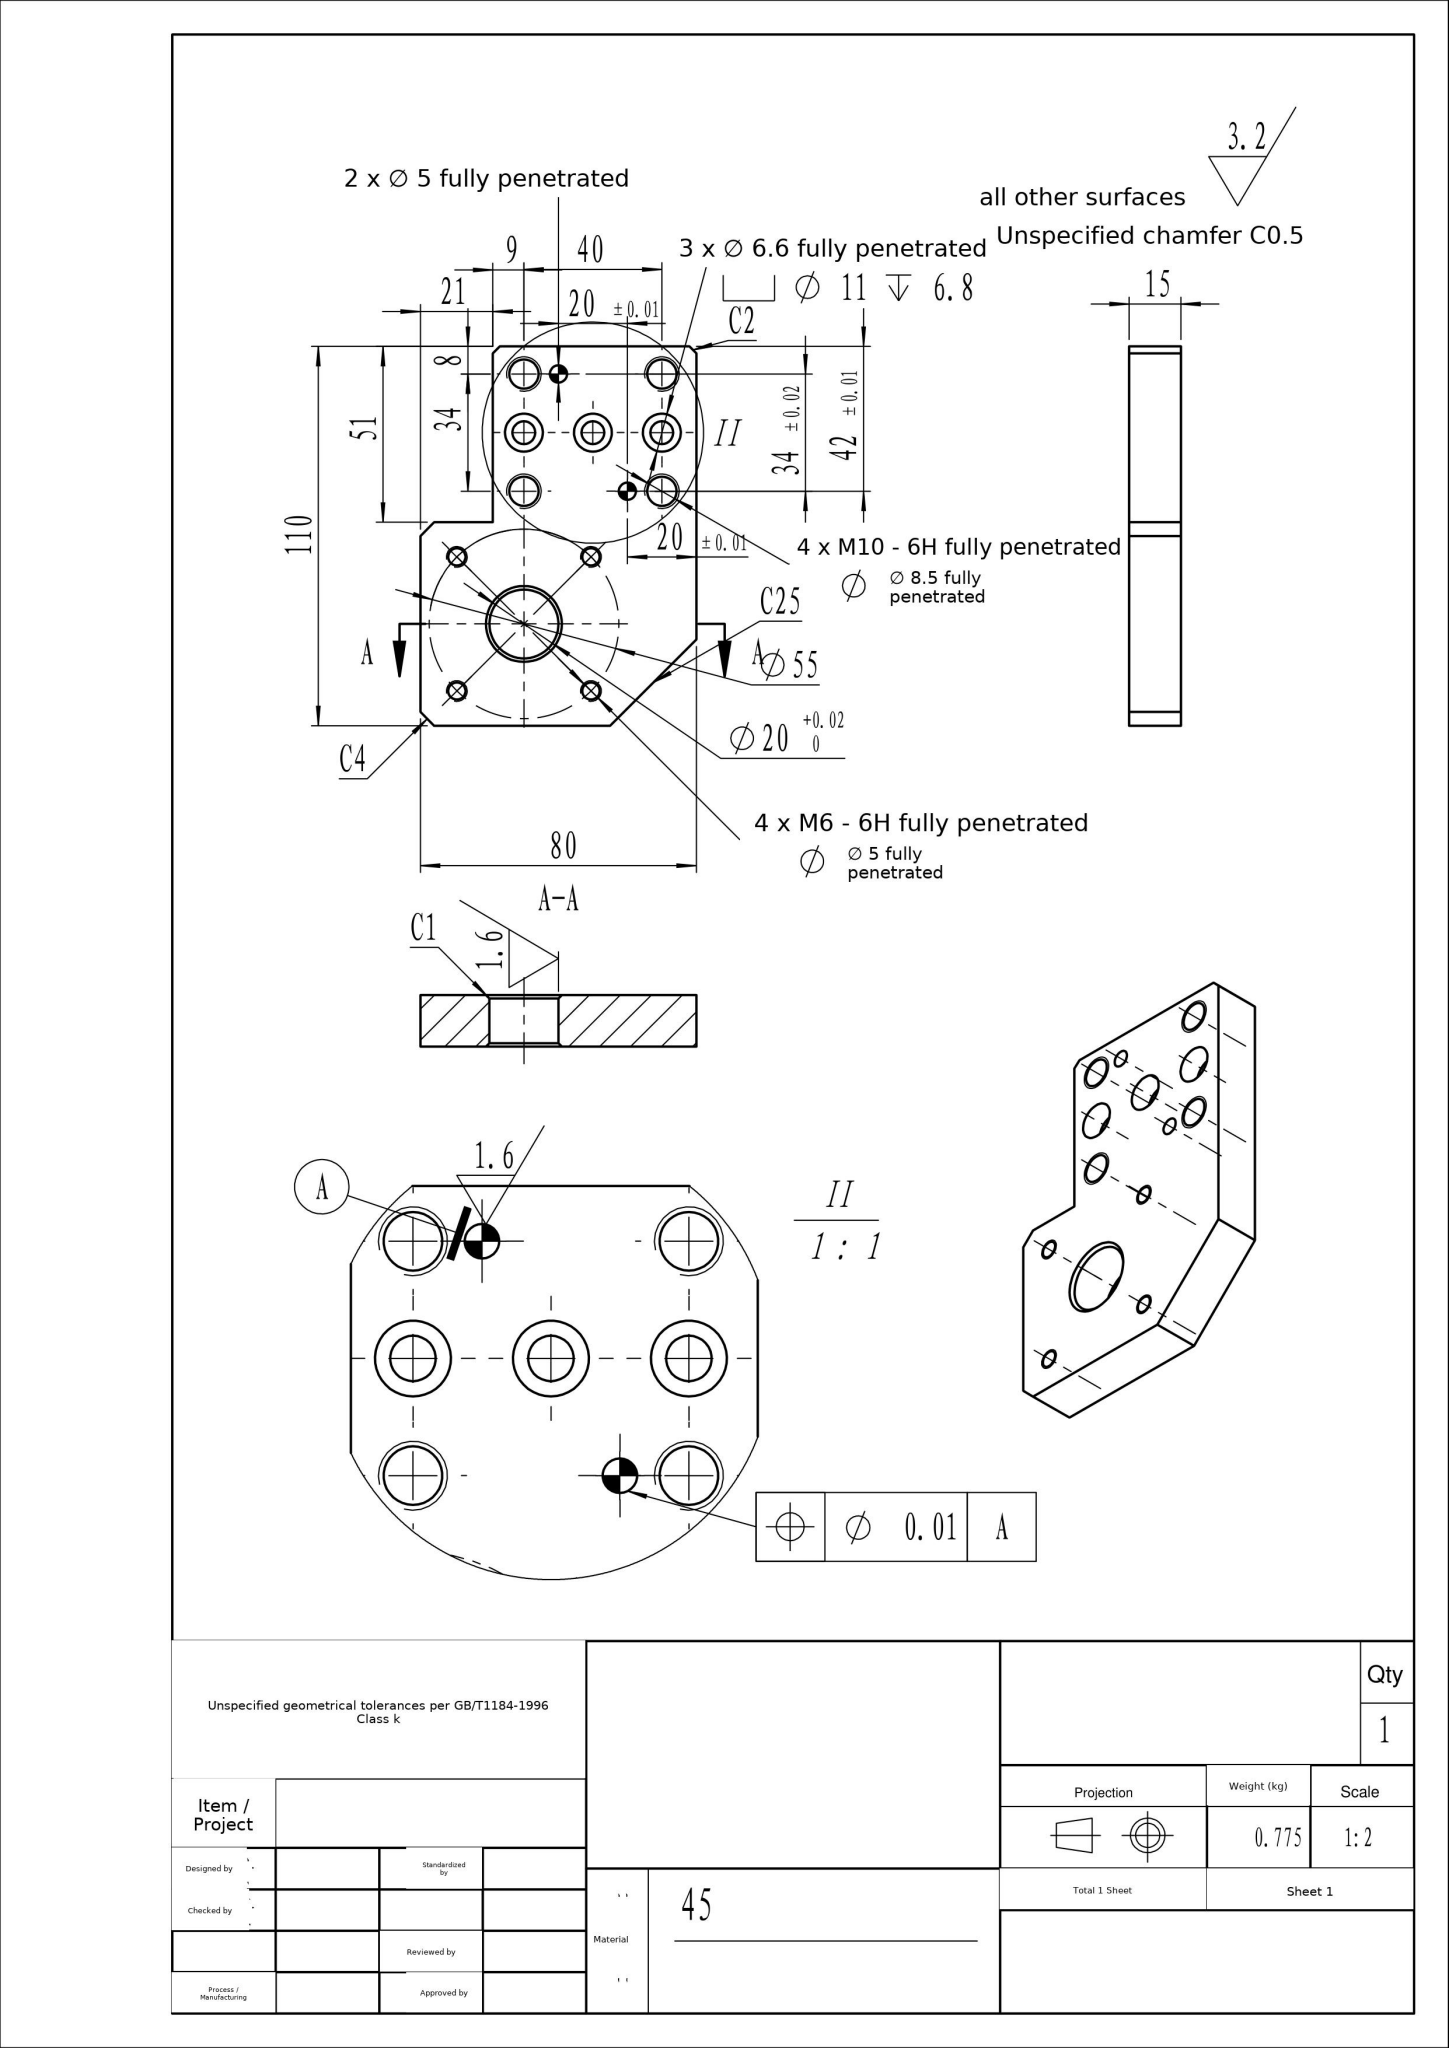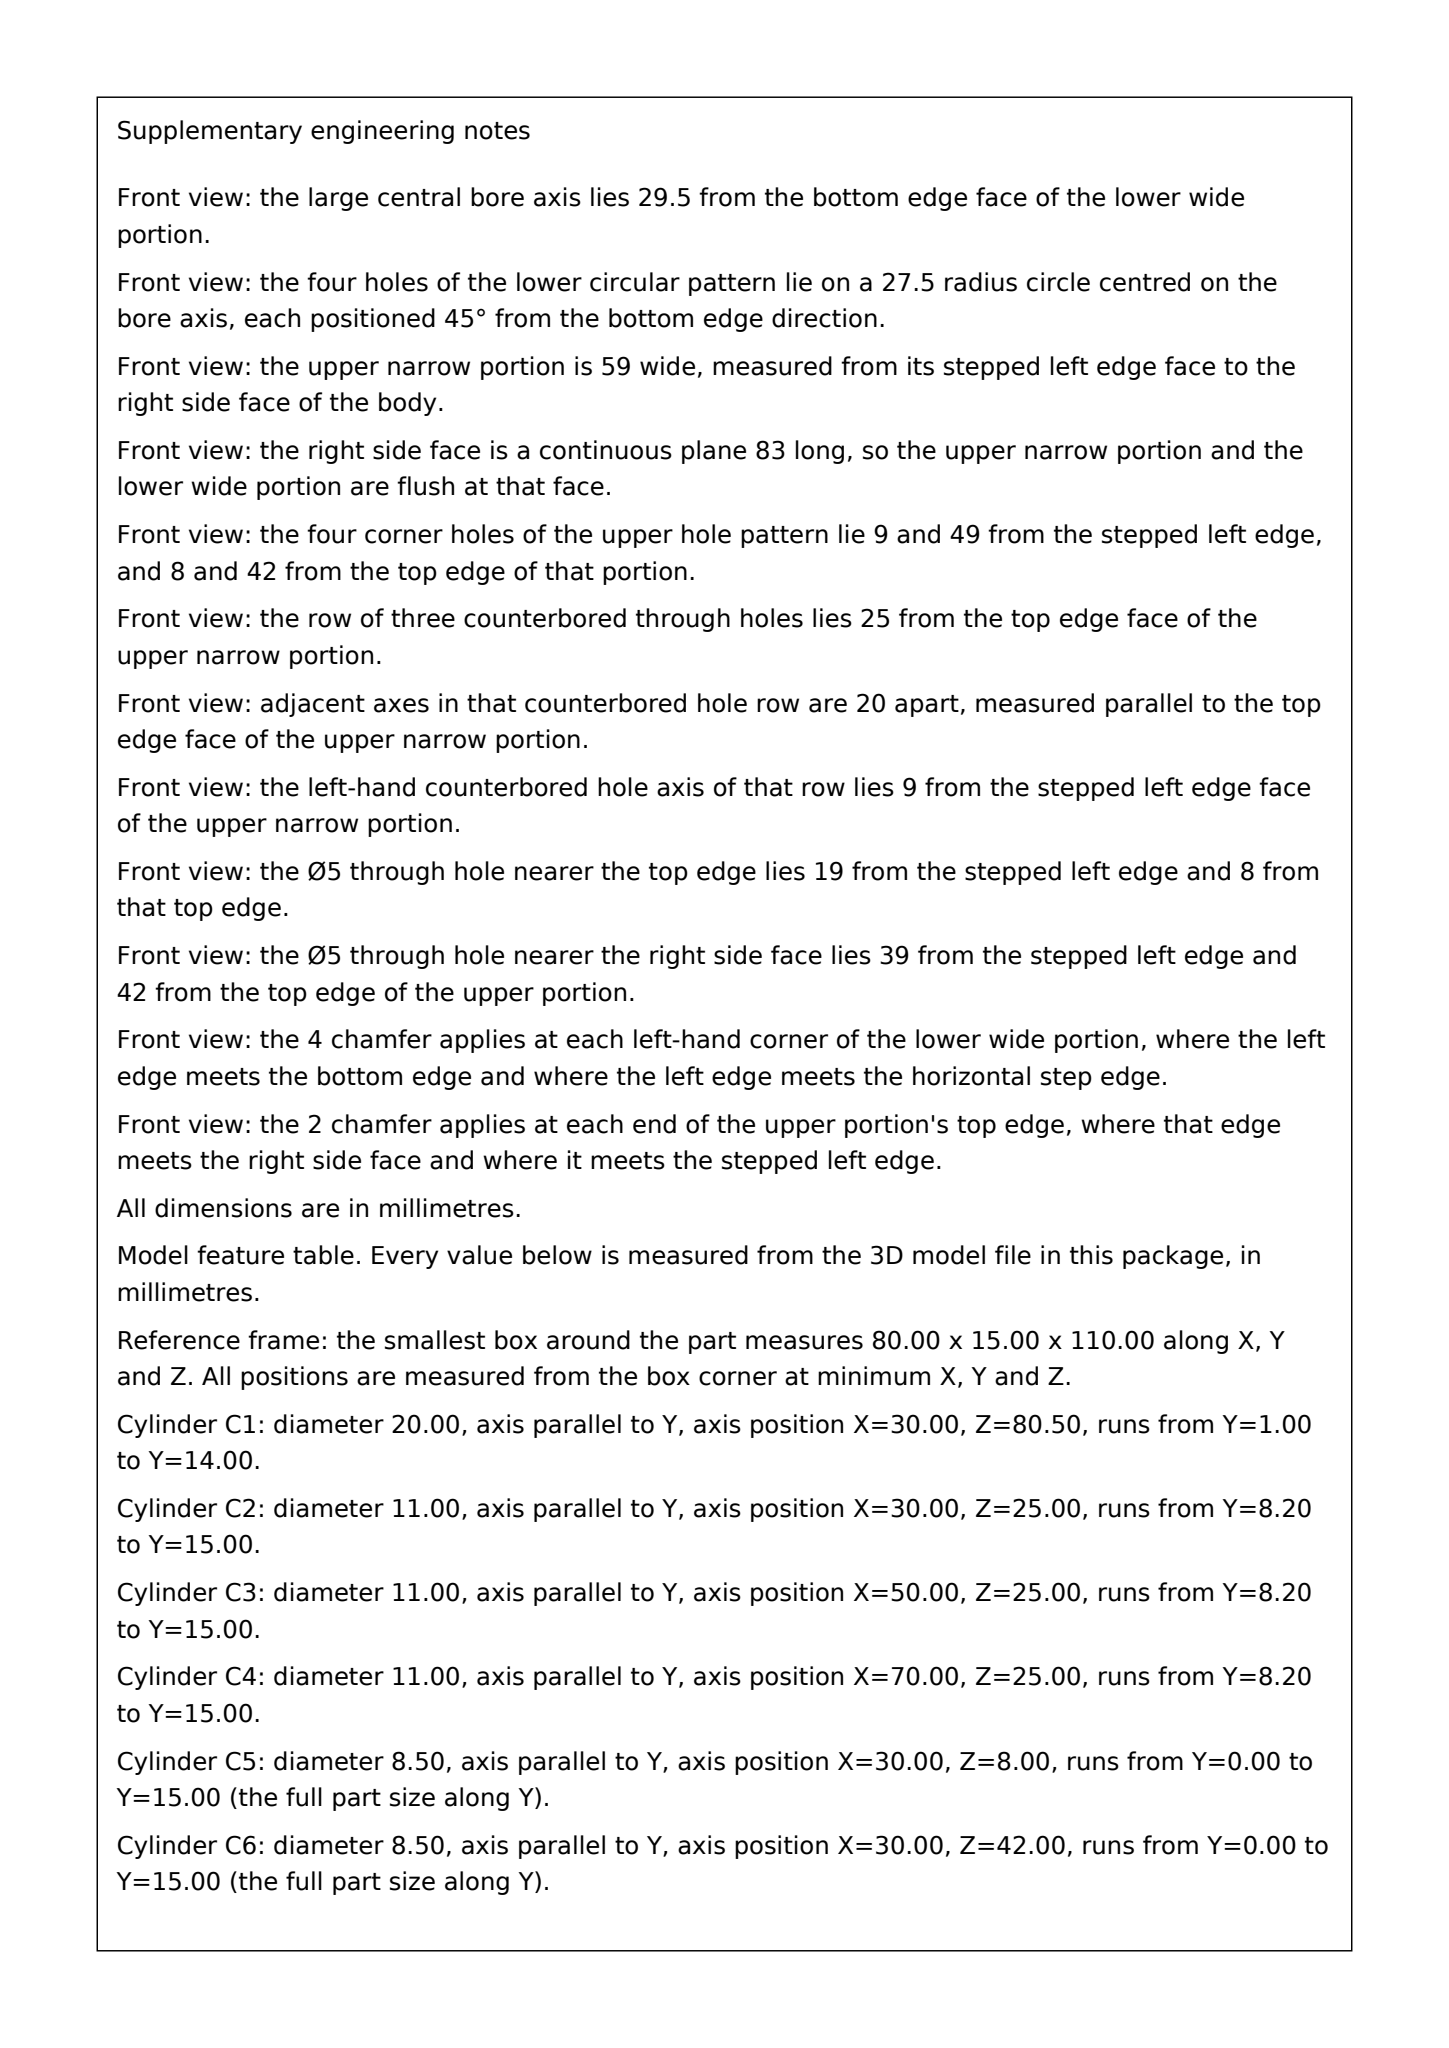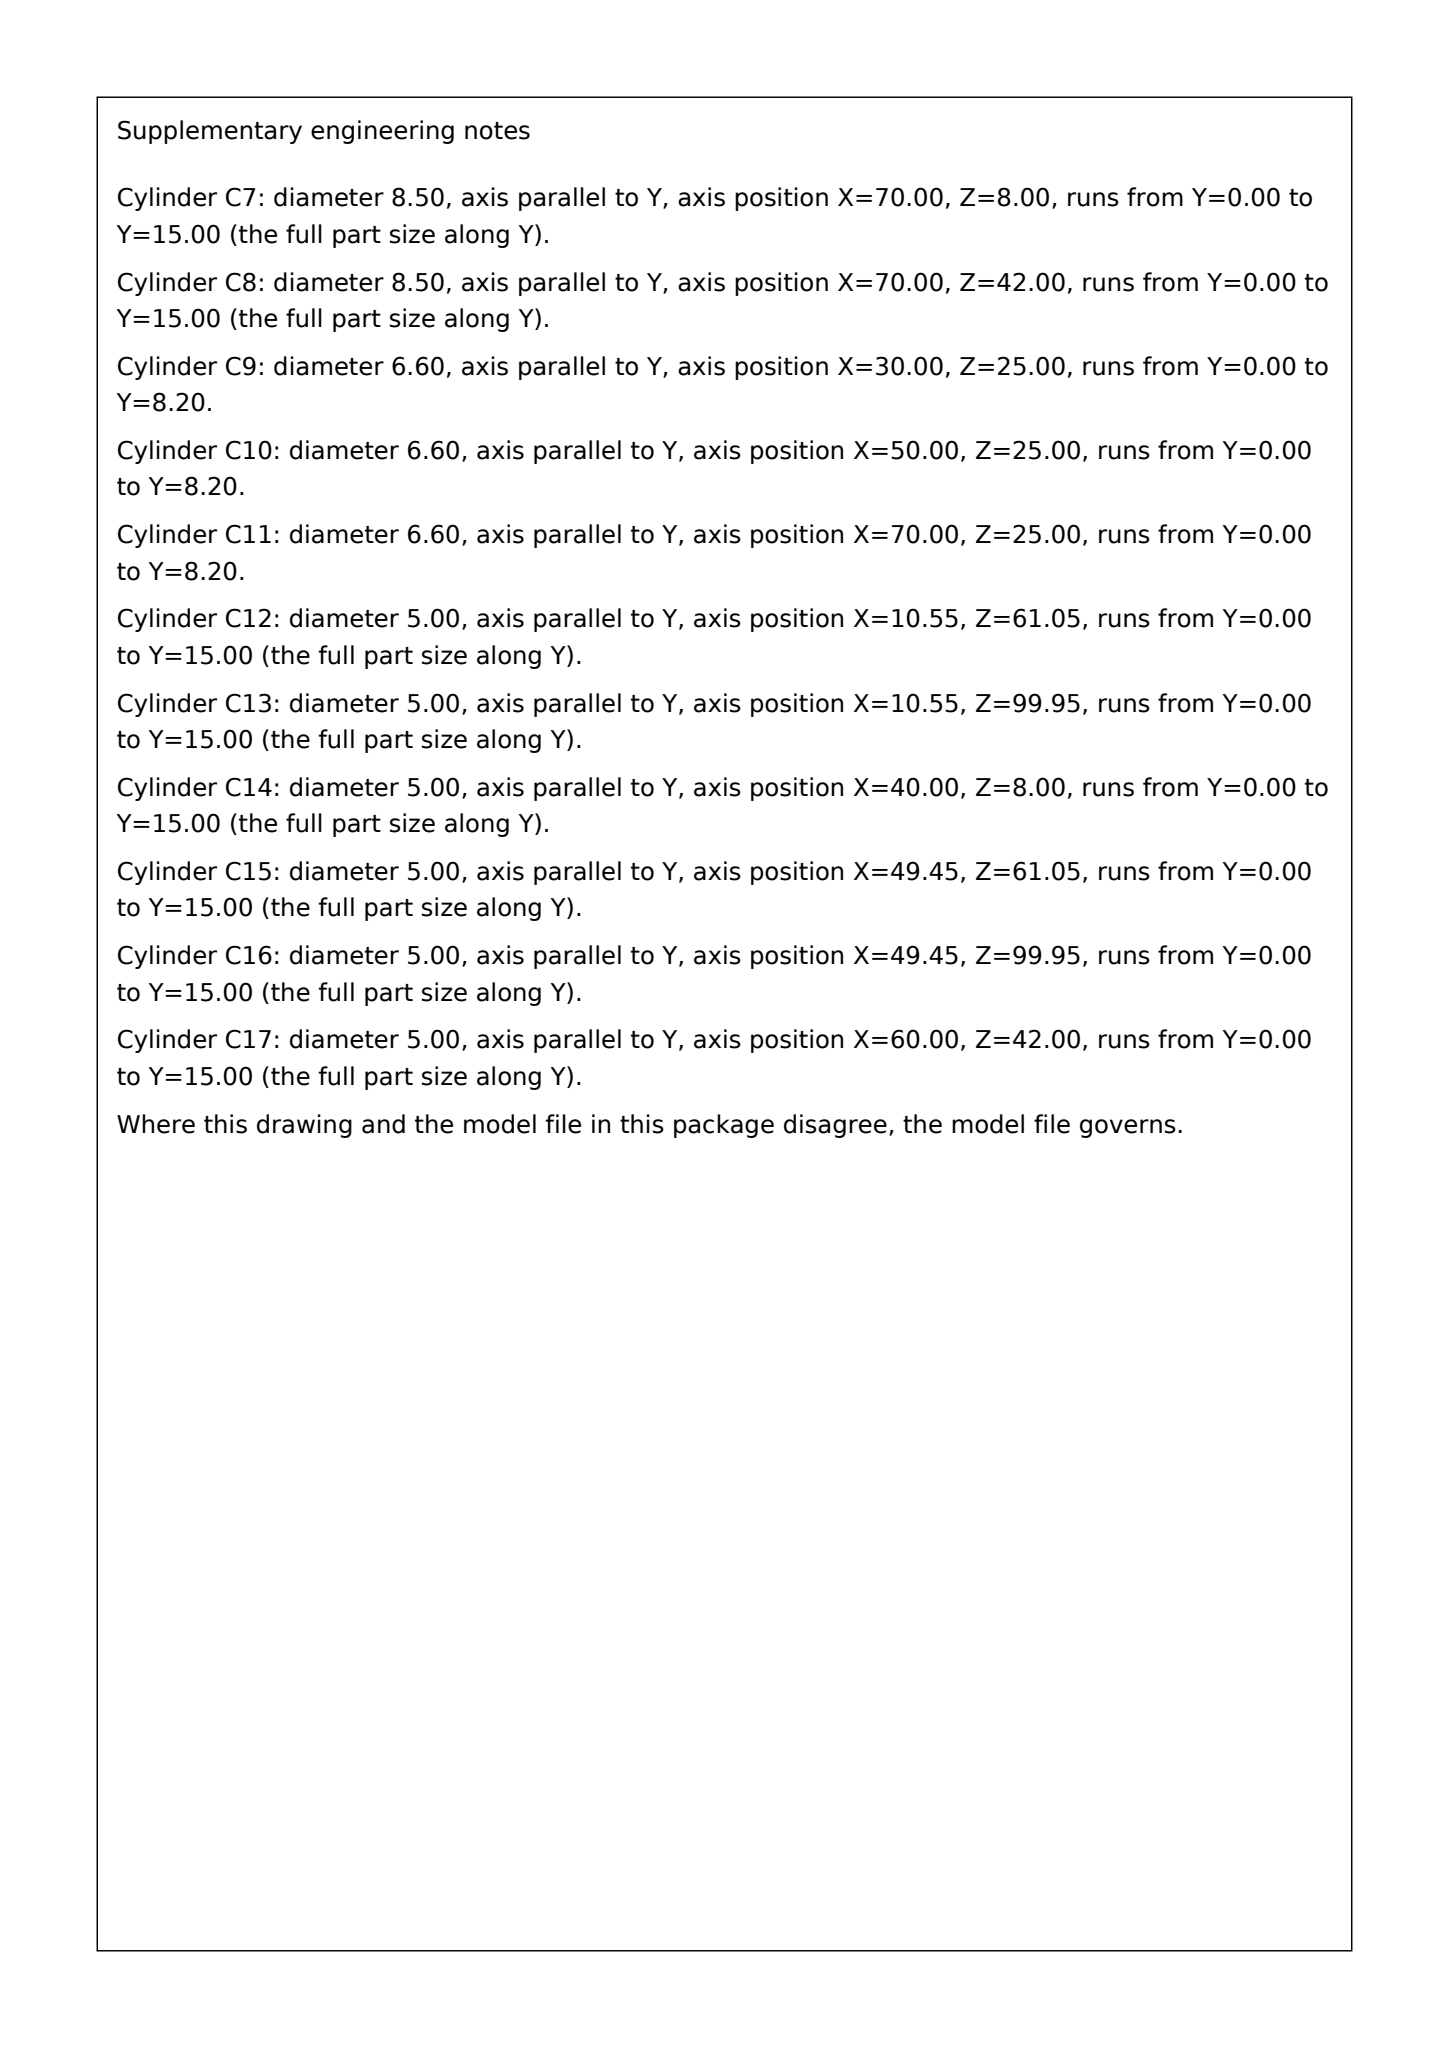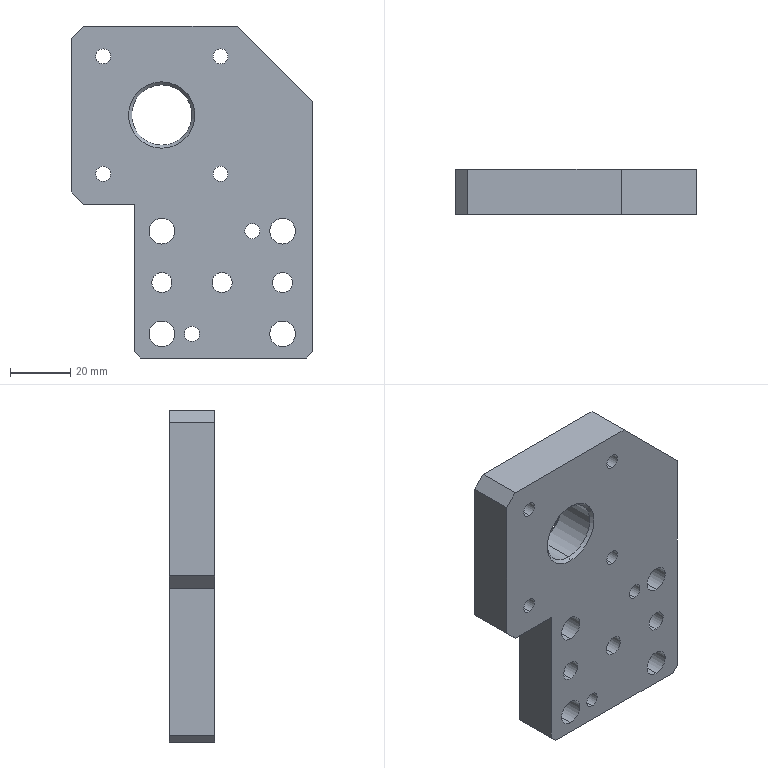Part | SolidWorks | mm | material 45 | 1 solid | 54 faces | box 80 x 15 x 110 mm | volume 98218 mm3 | cylinder 34 | plane 16 | cone 4 | commonest cylinder face diameters 5 x12 8.5 x8 11 x6 6.6 x6 20 x2
Drawing notes:
2 x Ø5 DOWEL: 40 & 60 FROM LH EDGE (AT Z=8 & Z=42 ROWS) | from the solid: Ø5.0 y-axis cyls at [40,null,8.0] and [60,null,42.0], L=15 thru; bbox X=80 from min corner
MIDDLE ROW 3 x Ø6.6/Ø11 C'BORE: 25 FROM TOP EDGE | from the solid: Ø6.6 & Ø11 cyls at z=25 (bbox z=0..110); drawing top edge = z=0, so 25 from top edge; rows at 8, 25, 42
4 x M6 EQL SP ON Ø55 B.C., 45° FROM CENTRELINES | from the solid: Ø5 holes at (10.55,61.05),(10.55,99.95),(49.45,61.05),(49.45,99.95) = ±19.45 from Ø20 center (30,80.5); R27.5, 45° spacing
build123d program:
from build123d import *

# Parameters (mm, degrees)
SKETCH1_W                                            = 80
SKETCH1_H                                            = 110
BOSS_EXTRUDE1_DEPTH                                  = 15
SKETCH2_W                                            = 21
SKETCH2_H                                            = 51
CUT_EXTRUDE1_DEPTH                                   = 70.642
SKETCH3_R                                            = 10
CUT_EXTRUDE2_DEPTH                                   = 70.642
CHAMFER1_SIZE                                        = 4
CHAMFER2_SIZE                                        = 2
CHAMFER3_SIZE                                        = 25
CHAMFER4_SIZE                                        = 1
M6_TAPPED_HOLE1_D                                    = 5
CIRPATTERN1_COUNT                                    = 4
M10_TAPPED_HOLE1_D                                   = 8.5
HOLE_SIZE_ACCORDING_TO_THE_TYPE_OF_HEXAG_D           = 6.6
HOLE_SIZE_ACCORDING_TO_THE_TYPE_OF_HEXAG_CBORE_D     = 11
HOLE_SIZE_ACCORDING_TO_THE_TYPE_OF_HEXAG_CBORE_DEPTH = 6.8
F_5_0_5_DIAMETER_HOLE1_D                             = 5


with BuildPart() as part:
    # Sketch1 → Boss-Extrude1 (new body)
    with BuildSketch(Plane(origin=(0, 0, 0), x_dir=(1, 0, 0), z_dir=(0, 1, 0))):
        Rectangle(SKETCH1_W, SKETCH1_H)
    extrude(amount=BOSS_EXTRUDE1_DEPTH)

    # Sketch2 → Cut-Extrude1 (cut, through all)
    with BuildSketch(Plane(origin=(0, 15, 0), x_dir=(1, 0, 0), z_dir=(0, 1, 0))):
        with Locations((-29.5, 29.5)):
            Rectangle(SKETCH2_W, SKETCH2_H)
    extrude(amount=-CUT_EXTRUDE1_DEPTH, mode=Mode.SUBTRACT)

    # Sketch3 → Cut-Extrude2 (cut, through all)
    with BuildSketch(Plane(origin=(0, 15, 0), x_dir=(1, 0, 0), z_dir=(0, 1, 0))):
        with Locations(Location((-10, -25.5, 0), (0, 0, 270))):
            Circle(SKETCH3_R)
    extrude(amount=-CUT_EXTRUDE2_DEPTH, mode=Mode.SUBTRACT)

    # Chamfer1
    chamfer1_edges = [part.edges().sort_by_distance(p)[0] for p in [
        (-40, 7.5, -4),
        (-40, 7.5, 55),
    ]]
    chamfer(chamfer1_edges, length=CHAMFER1_SIZE)

    # Chamfer2
    chamfer2_edges = [part.edges().sort_by_distance(p)[0] for p in [
        (-19, 7.5, -55),
        (40, 7.5, -55),
    ]]
    chamfer(chamfer2_edges, length=CHAMFER2_SIZE)

    # Chamfer3
    chamfer3_edges = [part.edges().sort_by_distance(p)[0] for p in [
        (40, 7.5, 55),
    ]]
    chamfer(chamfer3_edges, length=CHAMFER3_SIZE)

    # Chamfer4
    chamfer4_edges = [part.edges().sort_by_distance(p)[0] for p in [
        (-10, 0, 15.5),
        (-10, 15, 15.5),
    ]]
    chamfer(chamfer4_edges, length=CHAMFER4_SIZE)

    # M6 Tapped Hole1 (through all)
    with Locations(Plane(origin=(0, 15, 0), x_dir=(1, 0, 0), z_dir=(0, 1, 0))):
        with Locations((9.445, -6.055)):
            m6_tapped_hole1 = Hole(M6_TAPPED_HOLE1_D / 2)

    # CirPattern1: M6 Tapped Hole1 ×4 about axis
    cirpattern1_axis = Axis((-10, 0, 25.5), (0, 1, 0))
    for i in range(1, CIRPATTERN1_COUNT):
        add(m6_tapped_hole1.rotate(cirpattern1_axis, i * 360 / CIRPATTERN1_COUNT), mode=Mode.SUBTRACT)

    # M10 Tapped Hole1 (through all)
    with Locations(Plane(origin=(0, 15, 0), x_dir=(1, 0, 0), z_dir=(0, 1, 0))):
        with Locations((-10, 47), (30, 47), (30, 13), (-10, 13)):
            Hole(M10_TAPPED_HOLE1_D / 2)

    # Hole size according to the type of hexag (through all)
    with Locations(Plane(origin=(0, 15, 0), x_dir=(1, 0, 0), z_dir=(0, 1, 0))):
        with Locations((-10, 30), (10, 30), (30, 30)):
            CounterBoreHole(HOLE_SIZE_ACCORDING_TO_THE_TYPE_OF_HEXAG_D / 2, HOLE_SIZE_ACCORDING_TO_THE_TYPE_OF_HEXAG_CBORE_D / 2, HOLE_SIZE_ACCORDING_TO_THE_TYPE_OF_HEXAG_CBORE_DEPTH)

    # 5.0 _5_ Diameter Hole1 (through all)
    with Locations(Plane(origin=(0, 15, 0), x_dir=(1, 0, 0), z_dir=(0, 1, 0))):
        with Locations((0, 47), (20, 13)):
            Hole(F_5_0_5_DIAMETER_HOLE1_D / 2)


solid = part.part